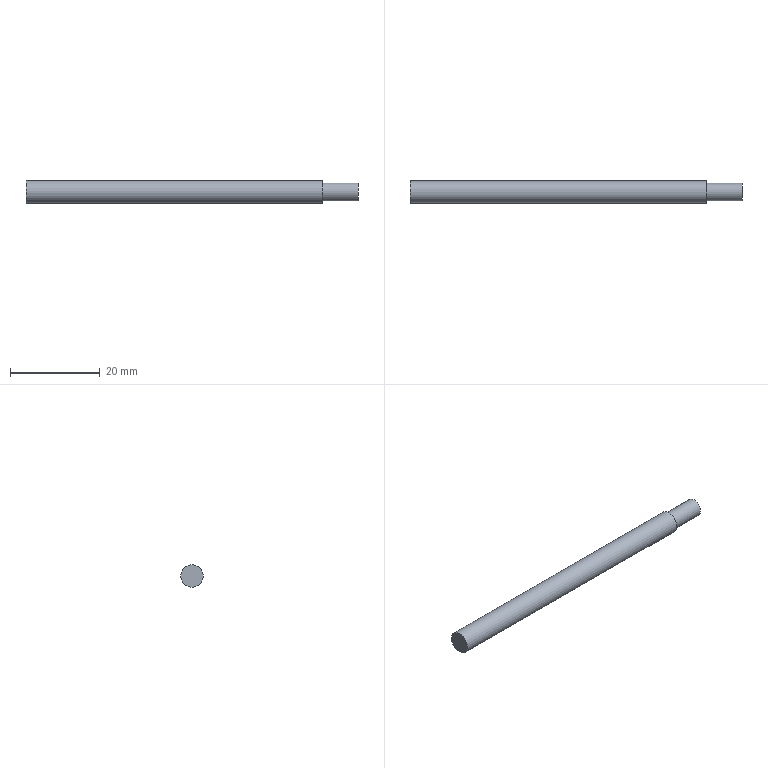Component | NX | PISTON_ROD_1 | 1 solid | 5 faces | box 74 x 5 x 5 mm | volume 1396 mm3 | plane 3 | cylinder 2 | commonest cylinder face diameters 5 x1 4 x1
STEP:
#1=CARTESIAN_POINT('',(0.,0.,0.));
#2=DIRECTION('',(0.,0.,1.));
#3=DIRECTION('',(1.,0.,0.));
#4=AXIS2_PLACEMENT_3D('',#1,#2,#3);
#5=CARTESIAN_POINT('',(86.201,-36.75,39.));
#6=VERTEX_POINT('',#5);
#7=CARTESIAN_POINT('',(86.201,-36.75,41.));
#8=DIRECTION('',(1.,0.,0.));
#9=DIRECTION('',(0.,0.,-1.));
#10=AXIS2_PLACEMENT_3D('',#7,#8,#9);
#11=CIRCLE('',#10,2.);
#12=CARTESIAN_POINT('',(86.201,-36.75,41.));
#13=DIRECTION('',(1.,0.,0.));
#14=DIRECTION('',(0.,0.,-1.));
#15=AXIS2_PLACEMENT_3D('',#12,#13,#14);
#16=PLANE('',#15);
#17=CARTESIAN_POINT('',(0.,0.));
#18=DIRECTION('',(1.,0.));
#19=AXIS2_PLACEMENT_2D('',#17,#18);
#20=CIRCLE('',#19,2.);
#21=(GEOMETRIC_REPRESENTATION_CONTEXT(2)PARAMETRIC_REPRESENTATION_CONTEXT()REPRESENTATION_CONTEXT('',''));
#22=DEFINITIONAL_REPRESENTATION('',(#20),#21);
#23=PCURVE('',#16,#22);
#24=CARTESIAN_POINT('',(86.201,-36.75,41.));
#25=DIRECTION('',(1.,0.,0.));
#26=DIRECTION('',(0.,0.,-1.));
#27=AXIS2_PLACEMENT_3D('',#24,#25,#26);
#28=CYLINDRICAL_SURFACE('',#27,2.);
#29=CARTESIAN_POINT('',(0.,0.));
#30=DIRECTION('',(1.,0.));
#31=VECTOR('',#30,1.);
#32=LINE('',#29,#31);
#33=(GEOMETRIC_REPRESENTATION_CONTEXT(2)PARAMETRIC_REPRESENTATION_CONTEXT()REPRESENTATION_CONTEXT('',''));
#34=DEFINITIONAL_REPRESENTATION('',(#32),#33);
#35=PCURVE('',#28,#34);
#36=SURFACE_CURVE('',#11,(#23,#35),.PCURVE_S1.);
#37=EDGE_CURVE('',#6,#6,#36,.T.);
#38=ORIENTED_EDGE('',*,*,#37,.F.);
#39=EDGE_LOOP('',(#38));
#40=FACE_BOUND('',#39,.T.);
#41=CARTESIAN_POINT('',(86.201,-36.75,38.5));
#42=VERTEX_POINT('',#41);
#43=CARTESIAN_POINT('',(86.201,-36.75,41.));
#44=DIRECTION('',(-1.,0.,0.));
#45=DIRECTION('',(0.,0.,-1.));
#46=AXIS2_PLACEMENT_3D('',#43,#44,#45);
#47=CIRCLE('',#46,2.5);
#48=CARTESIAN_POINT('',(2.5,0.));
#49=CARTESIAN_POINT('',(2.5,-4.33));
#50=CARTESIAN_POINT('',(-1.25,-2.165));
#51=CARTESIAN_POINT('',(-5.,-0.));
#52=CARTESIAN_POINT('',(-1.25,2.165));
#53=CARTESIAN_POINT('',(2.5,4.33));
#54=CARTESIAN_POINT('',(2.5,0.));
#55=(BOUNDED_CURVE()B_SPLINE_CURVE(2,(#48,#49,#50,#51,#52,#53,#54),.UNSPECIFIED.,.T.,.F.)B_SPLINE_CURVE_WITH_KNOTS((1,2,2,2,2,1),(-2.094,0.,2.094,4.189,6.283,8.378),.UNSPECIFIED.)CURVE()GEOMETRIC_REPRESENTATION_ITEM()RATIONAL_B_SPLINE_CURVE((1.,0.5,1.,0.5,1.,0.5,1.))REPRESENTATION_ITEM(''));
#56=(GEOMETRIC_REPRESENTATION_CONTEXT(2)PARAMETRIC_REPRESENTATION_CONTEXT()REPRESENTATION_CONTEXT('',''));
#57=DEFINITIONAL_REPRESENTATION('',(#55),#56);
#58=PCURVE('',#16,#57);
#59=CARTESIAN_POINT('',(20.201,-36.75,41.));
#60=DIRECTION('',(1.,0.,0.));
#61=DIRECTION('',(0.,0.,-1.));
#62=AXIS2_PLACEMENT_3D('',#59,#60,#61);
#63=CYLINDRICAL_SURFACE('',#62,2.5);
#64=CARTESIAN_POINT('',(6.283,66.));
#65=DIRECTION('',(-1.,0.));
#66=VECTOR('',#65,1.);
#67=LINE('',#64,#66);
#68=(GEOMETRIC_REPRESENTATION_CONTEXT(2)PARAMETRIC_REPRESENTATION_CONTEXT()REPRESENTATION_CONTEXT('',''));
#69=DEFINITIONAL_REPRESENTATION('',(#67),#68);
#70=PCURVE('',#63,#69);
#71=SURFACE_CURVE('',#47,(#58,#70),.PCURVE_S1.);
#72=EDGE_CURVE('',#42,#42,#71,.T.);
#73=ORIENTED_EDGE('',*,*,#72,.F.);
#74=EDGE_LOOP('',(#73));
#75=FACE_BOUND('',#74,.T.);
#76=ADVANCED_FACE('',(#40,#75),#16,.T.);
#77=CARTESIAN_POINT('',(20.201,-36.75,38.5));
#78=VERTEX_POINT('',#77);
#79=CARTESIAN_POINT('',(20.201,-36.75,41.));
#80=DIRECTION('',(1.,0.,0.));
#81=DIRECTION('',(0.,0.,-1.));
#82=AXIS2_PLACEMENT_3D('',#79,#80,#81);
#83=CIRCLE('',#82,2.5);
#84=CARTESIAN_POINT('',(20.201,-36.75,41.));
#85=DIRECTION('',(-1.,0.,0.));
#86=DIRECTION('',(0.,0.,1.));
#87=AXIS2_PLACEMENT_3D('',#84,#85,#86);
#88=PLANE('',#87);
#89=CARTESIAN_POINT('',(-2.5,0.));
#90=CARTESIAN_POINT('',(-2.5,4.33));
#91=CARTESIAN_POINT('',(1.25,2.165));
#92=CARTESIAN_POINT('',(5.,0.));
#93=CARTESIAN_POINT('',(1.25,-2.165));
#94=CARTESIAN_POINT('',(-2.5,-4.33));
#95=CARTESIAN_POINT('',(-2.5,0.));
#96=(BOUNDED_CURVE()B_SPLINE_CURVE(2,(#89,#90,#91,#92,#93,#94,#95),.UNSPECIFIED.,.T.,.F.)B_SPLINE_CURVE_WITH_KNOTS((1,2,2,2,2,1),(-2.094,0.,2.094,4.189,6.283,8.378),.UNSPECIFIED.)CURVE()GEOMETRIC_REPRESENTATION_ITEM()RATIONAL_B_SPLINE_CURVE((1.,0.5,1.,0.5,1.,0.5,1.))REPRESENTATION_ITEM(''));
#97=(GEOMETRIC_REPRESENTATION_CONTEXT(2)PARAMETRIC_REPRESENTATION_CONTEXT()REPRESENTATION_CONTEXT('',''));
#98=DEFINITIONAL_REPRESENTATION('',(#96),#97);
#99=PCURVE('',#88,#98);
#100=CARTESIAN_POINT('',(0.,0.));
#101=DIRECTION('',(1.,0.));
#102=VECTOR('',#101,1.);
#103=LINE('',#100,#102);
#104=(GEOMETRIC_REPRESENTATION_CONTEXT(2)PARAMETRIC_REPRESENTATION_CONTEXT()REPRESENTATION_CONTEXT('',''));
#105=DEFINITIONAL_REPRESENTATION('',(#103),#104);
#106=PCURVE('',#63,#105);
#107=SURFACE_CURVE('',#83,(#99,#106),.PCURVE_S1.);
#108=EDGE_CURVE('',#78,#78,#107,.T.);
#109=ORIENTED_EDGE('',*,*,#108,.F.);
#110=EDGE_LOOP('',(#109));
#111=FACE_BOUND('',#110,.T.);
#112=ADVANCED_FACE('',(#111),#88,.T.);
#113=ORIENTED_EDGE('',*,*,#72,.T.);
#114=CARTESIAN_POINT('',(20.201,-36.75,38.5));
#115=CARTESIAN_POINT('',(86.201,-36.75,38.5));
#116=B_SPLINE_CURVE_WITH_KNOTS('',1,(#114,#115),.UNSPECIFIED.,.F.,.F.,(2,2),(0.,66.),.PIECEWISE_BEZIER_KNOTS.);
#117=CARTESIAN_POINT('',(0.,0.));
#118=DIRECTION('',(0.,1.));
#119=VECTOR('',#118,1.);
#120=LINE('',#117,#119);
#121=(GEOMETRIC_REPRESENTATION_CONTEXT(2)PARAMETRIC_REPRESENTATION_CONTEXT()REPRESENTATION_CONTEXT('',''));
#122=DEFINITIONAL_REPRESENTATION('',(#120),#121);
#123=PCURVE('',#63,#122);
#124=CARTESIAN_POINT('',(6.283,0.));
#125=DIRECTION('',(0.,1.));
#126=VECTOR('',#125,1.);
#127=LINE('',#124,#126);
#128=(GEOMETRIC_REPRESENTATION_CONTEXT(2)PARAMETRIC_REPRESENTATION_CONTEXT()REPRESENTATION_CONTEXT('',''));
#129=DEFINITIONAL_REPRESENTATION('',(#127),#128);
#130=PCURVE('',#63,#129);
#131=SEAM_CURVE('',#116,(#123,#130),.PCURVE_S1.);
#132=EDGE_CURVE('',#78,#42,#131,.T.);
#133=ORIENTED_EDGE('',*,*,#132,.F.);
#134=ORIENTED_EDGE('',*,*,#108,.T.);
#135=ORIENTED_EDGE('',*,*,#132,.T.);
#136=EDGE_LOOP('',(#113,#133,#134,#135));
#137=FACE_BOUND('',#136,.T.);
#138=ADVANCED_FACE('',(#137),#63,.T.);
#139=CARTESIAN_POINT('',(94.201,-36.75,39.));
#140=VERTEX_POINT('',#139);
#141=CARTESIAN_POINT('',(94.201,-36.75,41.));
#142=DIRECTION('',(1.,0.,0.));
#143=DIRECTION('',(0.,0.,-1.));
#144=AXIS2_PLACEMENT_3D('',#141,#142,#143);
#145=CIRCLE('',#144,2.);
#146=CARTESIAN_POINT('',(94.201,-36.75,41.));
#147=DIRECTION('',(1.,0.,0.));
#148=DIRECTION('',(0.,0.,-1.));
#149=AXIS2_PLACEMENT_3D('',#146,#147,#148);
#150=PLANE('',#149);
#151=CARTESIAN_POINT('',(0.,0.));
#152=DIRECTION('',(1.,0.));
#153=AXIS2_PLACEMENT_2D('',#151,#152);
#154=CIRCLE('',#153,2.);
#155=(GEOMETRIC_REPRESENTATION_CONTEXT(2)PARAMETRIC_REPRESENTATION_CONTEXT()REPRESENTATION_CONTEXT('',''));
#156=DEFINITIONAL_REPRESENTATION('',(#154),#155);
#157=PCURVE('',#150,#156);
#158=CARTESIAN_POINT('',(0.,8.));
#159=DIRECTION('',(1.,0.));
#160=VECTOR('',#159,1.);
#161=LINE('',#158,#160);
#162=(GEOMETRIC_REPRESENTATION_CONTEXT(2)PARAMETRIC_REPRESENTATION_CONTEXT()REPRESENTATION_CONTEXT('',''));
#163=DEFINITIONAL_REPRESENTATION('',(#161),#162);
#164=PCURVE('',#28,#163);
#165=SURFACE_CURVE('',#145,(#157,#164),.PCURVE_S1.);
#166=EDGE_CURVE('',#140,#140,#165,.T.);
#167=ORIENTED_EDGE('',*,*,#166,.T.);
#168=EDGE_LOOP('',(#167));
#169=FACE_BOUND('',#168,.T.);
#170=ADVANCED_FACE('',(#169),#150,.T.);
#171=ORIENTED_EDGE('',*,*,#166,.F.);
#172=CARTESIAN_POINT('',(86.201,-36.75,39.));
#173=CARTESIAN_POINT('',(94.201,-36.75,39.));
#174=B_SPLINE_CURVE_WITH_KNOTS('',1,(#172,#173),.UNSPECIFIED.,.F.,.F.,(2,2),(0.,8.),.PIECEWISE_BEZIER_KNOTS.);
#175=CARTESIAN_POINT('',(0.,0.));
#176=DIRECTION('',(0.,1.));
#177=VECTOR('',#176,1.);
#178=LINE('',#175,#177);
#179=(GEOMETRIC_REPRESENTATION_CONTEXT(2)PARAMETRIC_REPRESENTATION_CONTEXT()REPRESENTATION_CONTEXT('',''));
#180=DEFINITIONAL_REPRESENTATION('',(#178),#179);
#181=PCURVE('',#28,#180);
#182=CARTESIAN_POINT('',(6.283,0.));
#183=DIRECTION('',(0.,1.));
#184=VECTOR('',#183,1.);
#185=LINE('',#182,#184);
#186=(GEOMETRIC_REPRESENTATION_CONTEXT(2)PARAMETRIC_REPRESENTATION_CONTEXT()REPRESENTATION_CONTEXT('',''));
#187=DEFINITIONAL_REPRESENTATION('',(#185),#186);
#188=PCURVE('',#28,#187);
#189=SEAM_CURVE('',#174,(#181,#188),.PCURVE_S1.);
#190=EDGE_CURVE('',#6,#140,#189,.T.);
#191=ORIENTED_EDGE('',*,*,#190,.F.);
#192=ORIENTED_EDGE('',*,*,#37,.T.);
#193=ORIENTED_EDGE('',*,*,#190,.T.);
#194=EDGE_LOOP('',(#171,#191,#192,#193));
#195=FACE_BOUND('',#194,.T.);
#196=ADVANCED_FACE('',(#195),#28,.T.);
#197=CLOSED_SHELL('',(#76,#112,#138,#170,#196));
#198=MANIFOLD_SOLID_BREP('',#197);
#199=(LENGTH_UNIT()NAMED_UNIT(*)SI_UNIT(.MILLI.,.METRE.));
#200=UNCERTAINTY_MEASURE_WITH_UNIT(LENGTH_MEASURE(0.00001),#199,'','');
#201=(NAMED_UNIT(*)PLANE_ANGLE_UNIT()SI_UNIT($,.RADIAN.));
#202=(NAMED_UNIT(*)SI_UNIT($,.STERADIAN.)SOLID_ANGLE_UNIT());
#203=(GEOMETRIC_REPRESENTATION_CONTEXT(3)GLOBAL_UNCERTAINTY_ASSIGNED_CONTEXT((#200))GLOBAL_UNIT_ASSIGNED_CONTEXT((#199,#201,#202))REPRESENTATION_CONTEXT('',''));
#204=ADVANCED_BREP_SHAPE_REPRESENTATION('',(#4,#198),#203);